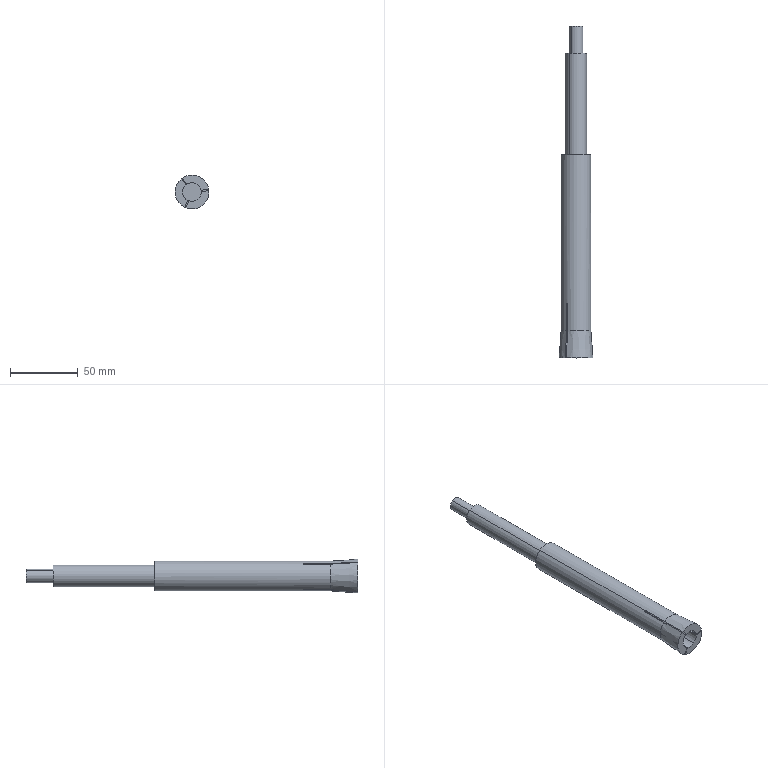Component | SolidWorks | HZ022-A001-D004-1 | 1 solid | 28 faces | box 25 x 245 x 25 mm | volume 51461 mm3 | plane 16 | cylinder 8 | cone 4 | commonest cylinder face diameters 10 x2 13.9 x2 22 x2 16 x2 | material S45C
STEP:
#1=COLOUR_RGB('',0.7922,0.8196,0.9333);
#2=FILL_AREA_STYLE_COLOUR('',#1);
#3=FILL_AREA_STYLE('',(#2));
#4=SURFACE_STYLE_FILL_AREA(#3);
#5=SURFACE_SIDE_STYLE('',(#4));
#6=SURFACE_STYLE_USAGE(.BOTH.,#5);
#7=PRESENTATION_STYLE_ASSIGNMENT((#6));
#8=CARTESIAN_POINT('',(-0.6243,0.2163,19.055));
#9=VERTEX_POINT('',#8);
#10=CARTESIAN_POINT('',(-0.3887,0.2163,18.74));
#11=VERTEX_POINT('',#10);
#12=CARTESIAN_POINT('',(-0.5065,0.2163,18.898));
#13=DIRECTION('',(0.,1.,0.));
#14=DIRECTION('',(-0.5984,0.,0.8012));
#15=AXIS2_PLACEMENT_3D('',#12,#13,#14);
#16=CIRCLE('',#15,0.1969);
#17=EDGE_CURVE('',#9,#11,#16,.T.);
#18=ORIENTED_EDGE('',*,*,#17,.T.);
#19=CARTESIAN_POINT('',(-0.3887,1.004,18.74));
#20=VERTEX_POINT('',#19);
#21=CARTESIAN_POINT('',(-0.3887,0.2163,18.74));
#22=DIRECTION('',(0.,1.,0.));
#23=VECTOR('',#22,39.37);
#24=LINE('',#21,#23);
#25=EDGE_CURVE('',#11,#20,#24,.T.);
#26=ORIENTED_EDGE('',*,*,#25,.T.);
#27=CARTESIAN_POINT('',(-0.6243,1.004,19.055));
#28=VERTEX_POINT('',#27);
#29=CARTESIAN_POINT('',(-0.5065,1.004,18.898));
#30=DIRECTION('',(0.,1.,0.));
#31=DIRECTION('',(-0.5984,0.,0.8012));
#32=AXIS2_PLACEMENT_3D('',#29,#30,#31);
#33=CIRCLE('',#32,0.1969);
#34=EDGE_CURVE('',#28,#20,#33,.T.);
#35=ORIENTED_EDGE('',*,*,#34,.F.);
#36=CARTESIAN_POINT('',(-0.6243,0.2163,19.055));
#37=DIRECTION('',(0.,1.,0.));
#38=VECTOR('',#37,39.37);
#39=LINE('',#36,#38);
#40=EDGE_CURVE('',#9,#28,#39,.T.);
#41=ORIENTED_EDGE('',*,*,#40,.F.);
#42=EDGE_LOOP('',(#18,#26,#35,#41));
#43=FACE_OUTER_BOUND('',#42,.T.);
#44=CARTESIAN_POINT('',(-0.5065,0.2163,18.898));
#45=DIRECTION('',(0.,1.,0.));
#46=DIRECTION('',(-0.5984,0.,0.8012));
#47=AXIS2_PLACEMENT_3D('',#44,#45,#46);
#48=CYLINDRICAL_SURFACE('',#47,0.1969);
#49=ADVANCED_FACE('',(#43),#48,.T.);
#50=CARTESIAN_POINT('',(-0.6702,-2.736,19.117));
#51=VERTEX_POINT('',#50);
#52=CARTESIAN_POINT('',(-0.3427,-2.736,18.678));
#53=VERTEX_POINT('',#52);
#54=CARTESIAN_POINT('',(-0.5065,-2.736,18.898));
#55=DIRECTION('',(0.,-1.,0.));
#56=DIRECTION('',(0.5984,0.,-0.8012));
#57=AXIS2_PLACEMENT_3D('',#54,#55,#56);
#58=CIRCLE('',#57,0.2736);
#59=EDGE_CURVE('',#51,#53,#58,.T.);
#60=ORIENTED_EDGE('',*,*,#59,.F.);
#61=CARTESIAN_POINT('',(-0.6702,-7.067,19.117));
#62=VERTEX_POINT('',#61);
#63=CARTESIAN_POINT('',(-0.6702,-2.736,19.117));
#64=DIRECTION('',(0.,-1.,0.));
#65=VECTOR('',#64,39.37);
#66=LINE('',#63,#65);
#67=EDGE_CURVE('',#51,#62,#66,.T.);
#68=ORIENTED_EDGE('',*,*,#67,.T.);
#69=CARTESIAN_POINT('',(-0.6856,-7.067,19.105));
#70=VERTEX_POINT('',#69);
#71=CARTESIAN_POINT('',(-0.5065,-7.067,18.898));
#72=DIRECTION('',(0.,1.,0.));
#73=DIRECTION('',(0.5984,0.,-0.8012));
#74=AXIS2_PLACEMENT_3D('',#71,#72,#73);
#75=CIRCLE('',#74,0.2736);
#76=EDGE_CURVE('',#70,#62,#75,.T.);
#77=ORIENTED_EDGE('',*,*,#76,.F.);
#78=CARTESIAN_POINT('',(-0.6856,-8.642,19.105));
#79=VERTEX_POINT('',#78);
#80=CARTESIAN_POINT('',(-0.6856,-2.736,19.105));
#81=DIRECTION('',(0.,-1.,0.));
#82=VECTOR('',#81,39.37);
#83=LINE('',#80,#82);
#84=EDGE_CURVE('',#70,#79,#83,.T.);
#85=ORIENTED_EDGE('',*,*,#84,.T.);
#86=CARTESIAN_POINT('',(-0.6323,-8.642,18.655));
#87=VERTEX_POINT('',#86);
#88=CARTESIAN_POINT('',(-0.5065,-8.642,18.898));
#89=DIRECTION('',(0.,-1.,0.));
#90=DIRECTION('',(0.5984,0.,-0.8012));
#91=AXIS2_PLACEMENT_3D('',#88,#89,#90);
#92=CIRCLE('',#91,0.2736);
#93=EDGE_CURVE('',#79,#87,#92,.T.);
#94=ORIENTED_EDGE('',*,*,#93,.T.);
#95=CARTESIAN_POINT('',(-0.6323,-7.067,18.655));
#96=VERTEX_POINT('',#95);
#97=CARTESIAN_POINT('',(-0.6323,-2.736,18.655));
#98=DIRECTION('',(0.,1.,0.));
#99=VECTOR('',#98,39.37);
#100=LINE('',#97,#99);
#101=EDGE_CURVE('',#87,#96,#100,.T.);
#102=ORIENTED_EDGE('',*,*,#101,.T.);
#103=CARTESIAN_POINT('',(-0.5961,-7.067,18.639));
#104=VERTEX_POINT('',#103);
#105=CARTESIAN_POINT('',(-0.5065,-7.067,18.898));
#106=DIRECTION('',(0.,1.,0.));
#107=DIRECTION('',(0.5984,0.,-0.8012));
#108=AXIS2_PLACEMENT_3D('',#105,#106,#107);
#109=CIRCLE('',#108,0.2736);
#110=EDGE_CURVE('',#104,#96,#109,.T.);
#111=ORIENTED_EDGE('',*,*,#110,.F.);
#112=CARTESIAN_POINT('',(-0.5961,-8.642,18.639));
#113=VERTEX_POINT('',#112);
#114=CARTESIAN_POINT('',(-0.5961,-2.736,18.639));
#115=DIRECTION('',(0.,-1.,0.));
#116=VECTOR('',#115,39.37);
#117=LINE('',#114,#116);
#118=EDGE_CURVE('',#104,#113,#117,.T.);
#119=ORIENTED_EDGE('',*,*,#118,.T.);
#120=CARTESIAN_POINT('',(-0.3427,-8.642,18.678));
#121=VERTEX_POINT('',#120);
#122=CARTESIAN_POINT('',(-0.5065,-8.642,18.898));
#123=DIRECTION('',(0.,-1.,0.));
#124=DIRECTION('',(0.5984,0.,-0.8012));
#125=AXIS2_PLACEMENT_3D('',#122,#123,#124);
#126=CIRCLE('',#125,0.2736);
#127=EDGE_CURVE('',#113,#121,#126,.T.);
#128=ORIENTED_EDGE('',*,*,#127,.T.);
#129=CARTESIAN_POINT('',(-0.3427,-2.736,18.678));
#130=DIRECTION('',(0.,-1.,0.));
#131=VECTOR('',#130,39.37);
#132=LINE('',#129,#131);
#133=EDGE_CURVE('',#53,#121,#132,.T.);
#134=ORIENTED_EDGE('',*,*,#133,.F.);
#135=EDGE_LOOP('',(#60,#68,#77,#85,#94,#102,#111,#119,#128,#134));
#136=FACE_OUTER_BOUND('',#135,.T.);
#137=CARTESIAN_POINT('',(-0.5065,-2.736,18.898));
#138=DIRECTION('',(0.,-1.,0.));
#139=DIRECTION('',(0.5984,0.,-0.8012));
#140=AXIS2_PLACEMENT_3D('',#137,#138,#139);
#141=CYLINDRICAL_SURFACE('',#140,0.2736);
#142=ADVANCED_FACE('',(#136),#141,.F.);
#143=CARTESIAN_POINT('',(-0.07456,-7.855,18.929));
#144=VERTEX_POINT('',#143);
#145=CARTESIAN_POINT('',(-0.2473,-7.855,18.551));
#146=VERTEX_POINT('',#145);
#147=CARTESIAN_POINT('',(-0.5065,-7.855,18.898));
#148=DIRECTION('',(0.,1.,0.));
#149=DIRECTION('',(-0.5984,0.,0.8012));
#150=AXIS2_PLACEMENT_3D('',#147,#148,#149);
#151=CIRCLE('',#150,0.4331);
#152=EDGE_CURVE('',#144,#146,#151,.T.);
#153=ORIENTED_EDGE('',*,*,#152,.T.);
#154=CARTESIAN_POINT('',(-0.2473,-2.736,18.551));
#155=VERTEX_POINT('',#154);
#156=CARTESIAN_POINT('',(-0.2473,-2.736,18.551));
#157=DIRECTION('',(0.,1.,0.));
#158=VECTOR('',#157,39.37);
#159=LINE('',#156,#158);
#160=EDGE_CURVE('',#146,#155,#159,.T.);
#161=ORIENTED_EDGE('',*,*,#160,.T.);
#162=CARTESIAN_POINT('',(-0.7657,-2.736,19.245));
#163=VERTEX_POINT('',#162);
#164=CARTESIAN_POINT('',(-0.5065,-2.736,18.898));
#165=DIRECTION('',(0.,1.,0.));
#166=DIRECTION('',(-0.5984,0.,0.8012));
#167=AXIS2_PLACEMENT_3D('',#164,#165,#166);
#168=CIRCLE('',#167,0.4331);
#169=EDGE_CURVE('',#163,#155,#168,.T.);
#170=ORIENTED_EDGE('',*,*,#169,.F.);
#171=CARTESIAN_POINT('',(-0.7657,-7.067,19.245));
#172=VERTEX_POINT('',#171);
#173=CARTESIAN_POINT('',(-0.7657,-2.736,19.245));
#174=DIRECTION('',(0.,1.,0.));
#175=VECTOR('',#174,39.37);
#176=LINE('',#173,#175);
#177=EDGE_CURVE('',#172,#163,#176,.T.);
#178=ORIENTED_EDGE('',*,*,#177,.F.);
#179=CARTESIAN_POINT('',(-0.7496,-7.067,19.256));
#180=VERTEX_POINT('',#179);
#181=CARTESIAN_POINT('',(-0.5065,-7.067,18.898));
#182=DIRECTION('',(0.,1.,0.));
#183=DIRECTION('',(0.5984,0.,-0.8012));
#184=AXIS2_PLACEMENT_3D('',#181,#182,#183);
#185=CIRCLE('',#184,0.4331);
#186=EDGE_CURVE('',#172,#180,#185,.T.);
#187=ORIENTED_EDGE('',*,*,#186,.T.);
#188=CARTESIAN_POINT('',(-0.7496,-7.855,19.256));
#189=VERTEX_POINT('',#188);
#190=CARTESIAN_POINT('',(-0.7496,-2.736,19.256));
#191=DIRECTION('',(0.,1.,0.));
#192=VECTOR('',#191,39.37);
#193=LINE('',#190,#192);
#194=EDGE_CURVE('',#189,#180,#193,.T.);
#195=ORIENTED_EDGE('',*,*,#194,.F.);
#196=CARTESIAN_POINT('',(-0.07919,-7.855,18.968));
#197=VERTEX_POINT('',#196);
#198=CARTESIAN_POINT('',(-0.5065,-7.855,18.898));
#199=DIRECTION('',(0.,1.,0.));
#200=DIRECTION('',(-0.5984,0.,0.8012));
#201=AXIS2_PLACEMENT_3D('',#198,#199,#200);
#202=CIRCLE('',#201,0.4331);
#203=EDGE_CURVE('',#189,#197,#202,.T.);
#204=ORIENTED_EDGE('',*,*,#203,.T.);
#205=CARTESIAN_POINT('',(-0.07919,-7.067,18.968));
#206=VERTEX_POINT('',#205);
#207=CARTESIAN_POINT('',(-0.07919,-2.736,18.968));
#208=DIRECTION('',(0.,-1.,0.));
#209=VECTOR('',#208,39.37);
#210=LINE('',#207,#209);
#211=EDGE_CURVE('',#206,#197,#210,.T.);
#212=ORIENTED_EDGE('',*,*,#211,.F.);
#213=CARTESIAN_POINT('',(-0.07456,-7.067,18.929));
#214=VERTEX_POINT('',#213);
#215=CARTESIAN_POINT('',(-0.5065,-7.067,18.898));
#216=DIRECTION('',(0.,1.,0.));
#217=DIRECTION('',(0.5984,0.,-0.8012));
#218=AXIS2_PLACEMENT_3D('',#215,#216,#217);
#219=CIRCLE('',#218,0.4331);
#220=EDGE_CURVE('',#206,#214,#219,.T.);
#221=ORIENTED_EDGE('',*,*,#220,.T.);
#222=CARTESIAN_POINT('',(-0.07456,-2.736,18.929));
#223=DIRECTION('',(0.,1.,0.));
#224=VECTOR('',#223,39.37);
#225=LINE('',#222,#224);
#226=EDGE_CURVE('',#144,#214,#225,.T.);
#227=ORIENTED_EDGE('',*,*,#226,.F.);
#228=EDGE_LOOP('',(#153,#161,#170,#178,#187,#195,#204,#212,#221,#227));
#229=FACE_OUTER_BOUND('',#228,.T.);
#230=CARTESIAN_POINT('',(-0.5065,-2.736,18.898));
#231=DIRECTION('',(0.,1.,0.));
#232=DIRECTION('',(-0.5984,0.,0.8012));
#233=AXIS2_PLACEMENT_3D('',#230,#231,#232);
#234=CYLINDRICAL_SURFACE('',#233,0.4331);
#235=ADVANCED_FACE('',(#229),#234,.T.);
#236=CARTESIAN_POINT('',(-0.6591,-7.855,18.492));
#237=VERTEX_POINT('',#236);
#238=CARTESIAN_POINT('',(-0.5065,-7.855,18.898));
#239=DIRECTION('',(0.,1.,0.));
#240=DIRECTION('',(-0.5984,0.,0.8012));
#241=AXIS2_PLACEMENT_3D('',#238,#239,#240);
#242=CIRCLE('',#241,0.4331);
#243=EDGE_CURVE('',#146,#237,#242,.T.);
#244=ORIENTED_EDGE('',*,*,#243,.F.);
#245=CARTESIAN_POINT('',(-0.212,-8.642,18.503));
#246=VERTEX_POINT('',#245);
#247=CARTESIAN_POINT('',(-0.2473,-7.855,18.551));
#248=DIRECTION('',(0.04476,-0.9972,-0.05992));
#249=VECTOR('',#248,39.37);
#250=LINE('',#247,#249);
#251=EDGE_CURVE('',#146,#246,#250,.T.);
#252=ORIENTED_EDGE('',*,*,#251,.T.);
#253=CARTESIAN_POINT('',(-0.6824,-8.642,18.438));
#254=VERTEX_POINT('',#253);
#255=CARTESIAN_POINT('',(-0.5065,-8.642,18.898));
#256=DIRECTION('',(0.,1.,0.));
#257=DIRECTION('',(-0.5984,0.,0.8012));
#258=AXIS2_PLACEMENT_3D('',#255,#256,#257);
#259=CIRCLE('',#258,0.4921);
#260=EDGE_CURVE('',#246,#254,#259,.T.);
#261=ORIENTED_EDGE('',*,*,#260,.T.);
#262=CARTESIAN_POINT('',(-0.6591,-7.855,18.492));
#263=CARTESIAN_POINT('',(-0.6669,-8.117,18.474));
#264=CARTESIAN_POINT('',(-0.6747,-8.379,18.456));
#265=CARTESIAN_POINT('',(-0.6824,-8.642,18.438));
#266=B_SPLINE_CURVE_WITH_KNOTS('',3,(#262,#263,#264,#265),.UNSPECIFIED.,.F.,.F.,(4,4),(0.0000002,0.02006),.UNSPECIFIED.);
#267=EDGE_CURVE('',#237,#254,#266,.T.);
#268=ORIENTED_EDGE('',*,*,#267,.F.);
#269=EDGE_LOOP('',(#244,#252,#261,#268));
#270=FACE_OUTER_BOUND('',#269,.T.);
#271=CARTESIAN_POINT('',(-0.5065,-7.855,18.898));
#272=DIRECTION('',(0.,-1.,0.));
#273=DIRECTION('',(0.5984,0.,-0.8012));
#274=AXIS2_PLACEMENT_3D('',#271,#272,#273);
#275=CONICAL_SURFACE('',#274,0.4331,0.07486);
#276=ADVANCED_FACE('',(#270),#275,.T.);
#277=CARTESIAN_POINT('',(-0.695,0.2163,19.15));
#278=VERTEX_POINT('',#277);
#279=CARTESIAN_POINT('',(-0.318,0.2163,18.645));
#280=VERTEX_POINT('',#279);
#281=CARTESIAN_POINT('',(-0.5065,0.2163,18.898));
#282=DIRECTION('',(0.,1.,0.));
#283=DIRECTION('',(-0.5984,0.,0.8012));
#284=AXIS2_PLACEMENT_3D('',#281,#282,#283);
#285=CIRCLE('',#284,0.315);
#286=EDGE_CURVE('',#278,#280,#285,.T.);
#287=ORIENTED_EDGE('',*,*,#286,.F.);
#288=CARTESIAN_POINT('',(-0.695,-2.736,19.15));
#289=VERTEX_POINT('',#288);
#290=CARTESIAN_POINT('',(-0.695,1.004,19.15));
#291=DIRECTION('',(0.,-1.,0.));
#292=VECTOR('',#291,39.37);
#293=LINE('',#290,#292);
#294=EDGE_CURVE('',#278,#289,#293,.T.);
#295=ORIENTED_EDGE('',*,*,#294,.T.);
#296=CARTESIAN_POINT('',(-0.318,-2.736,18.645));
#297=VERTEX_POINT('',#296);
#298=CARTESIAN_POINT('',(-0.5065,-2.736,18.898));
#299=DIRECTION('',(0.,1.,0.));
#300=DIRECTION('',(-0.5984,0.,0.8012));
#301=AXIS2_PLACEMENT_3D('',#298,#299,#300);
#302=CIRCLE('',#301,0.315);
#303=EDGE_CURVE('',#289,#297,#302,.T.);
#304=ORIENTED_EDGE('',*,*,#303,.T.);
#305=CARTESIAN_POINT('',(-0.318,1.004,18.645));
#306=DIRECTION('',(0.,-1.,0.));
#307=VECTOR('',#306,39.37);
#308=LINE('',#305,#307);
#309=EDGE_CURVE('',#280,#297,#308,.T.);
#310=ORIENTED_EDGE('',*,*,#309,.F.);
#311=EDGE_LOOP('',(#287,#295,#304,#310));
#312=FACE_OUTER_BOUND('',#311,.T.);
#313=CARTESIAN_POINT('',(-0.5065,1.004,18.898));
#314=DIRECTION('',(0.,-1.,0.));
#315=DIRECTION('',(0.5984,0.,-0.8012));
#316=AXIS2_PLACEMENT_3D('',#313,#314,#315);
#317=CYLINDRICAL_SURFACE('',#316,0.315);
#318=ADVANCED_FACE('',(#312),#317,.T.);
#319=ORIENTED_EDGE('',*,*,#294,.F.);
#320=CARTESIAN_POINT('',(-0.5065,0.2163,18.898));
#321=DIRECTION('',(0.,1.,0.));
#322=DIRECTION('',(-0.5984,0.,0.8012));
#323=AXIS2_PLACEMENT_3D('',#320,#321,#322);
#324=CIRCLE('',#323,0.315);
#325=EDGE_CURVE('',#280,#278,#324,.T.);
#326=ORIENTED_EDGE('',*,*,#325,.F.);
#327=ORIENTED_EDGE('',*,*,#309,.T.);
#328=CARTESIAN_POINT('',(-0.5065,-2.736,18.898));
#329=DIRECTION('',(0.,1.,0.));
#330=DIRECTION('',(-0.5984,0.,0.8012));
#331=AXIS2_PLACEMENT_3D('',#328,#329,#330);
#332=CIRCLE('',#331,0.315);
#333=EDGE_CURVE('',#297,#289,#332,.T.);
#334=ORIENTED_EDGE('',*,*,#333,.T.);
#335=EDGE_LOOP('',(#319,#326,#327,#334));
#336=FACE_OUTER_BOUND('',#335,.T.);
#337=CARTESIAN_POINT('',(-0.5065,1.004,18.898));
#338=DIRECTION('',(0.,-1.,0.));
#339=DIRECTION('',(0.5984,0.,-0.8012));
#340=AXIS2_PLACEMENT_3D('',#337,#338,#339);
#341=CYLINDRICAL_SURFACE('',#340,0.315);
#342=ADVANCED_FACE('',(#336),#341,.T.);
#343=CARTESIAN_POINT('',(-0.7186,-8.642,18.454));
#344=VERTEX_POINT('',#343);
#345=CARTESIAN_POINT('',(-0.9263,-8.642,17.97));
#346=DIRECTION('',(-0.3946,0.,-0.9188));
#347=VECTOR('',#346,39.37);
#348=LINE('',#345,#347);
#349=EDGE_CURVE('',#87,#344,#348,.T.);
#350=ORIENTED_EDGE('',*,*,#349,.F.);
#351=ORIENTED_EDGE('',*,*,#93,.F.);
#352=CARTESIAN_POINT('',(-0.8165,-8.642,19.28));
#353=VERTEX_POINT('',#352);
#354=CARTESIAN_POINT('',(-1.131,-8.642,19.701));
#355=DIRECTION('',(0.5984,0.,-0.8012));
#356=VECTOR('',#355,39.37);
#357=LINE('',#354,#356);
#358=EDGE_CURVE('',#353,#79,#357,.T.);
#359=ORIENTED_EDGE('',*,*,#358,.F.);
#360=CARTESIAN_POINT('',(-0.5065,-8.642,18.898));
#361=DIRECTION('',(0.,1.,0.));
#362=DIRECTION('',(-0.5984,0.,0.8012));
#363=AXIS2_PLACEMENT_3D('',#360,#361,#362);
#364=CIRCLE('',#363,0.4921);
#365=EDGE_CURVE('',#344,#353,#364,.T.);
#366=ORIENTED_EDGE('',*,*,#365,.F.);
#367=EDGE_LOOP('',(#350,#351,#359,#366));
#368=FACE_OUTER_BOUND('',#367,.T.);
#369=CARTESIAN_POINT('',(-0.5065,-8.642,18.898));
#370=DIRECTION('',(0.,-1.,0.));
#371=DIRECTION('',(0.5984,0.,-0.8012));
#372=AXIS2_PLACEMENT_3D('',#369,#370,#371);
#373=PLANE('',#372);
#374=ADVANCED_FACE('',(#368),#373,.T.);
#375=CARTESIAN_POINT('',(-0.0205,-8.642,18.975));
#376=VERTEX_POINT('',#375);
#377=CARTESIAN_POINT('',(-0.2378,-8.642,18.949));
#378=VERTEX_POINT('',#377);
#379=CARTESIAN_POINT('',(0.5021,-8.642,19.037));
#380=DIRECTION('',(-0.9931,0.,-0.1177));
#381=VECTOR('',#380,39.37);
#382=LINE('',#379,#381);
#383=EDGE_CURVE('',#376,#378,#382,.T.);
#384=ORIENTED_EDGE('',*,*,#383,.F.);
#385=CARTESIAN_POINT('',(-0.785,-8.642,19.303));
#386=VERTEX_POINT('',#385);
#387=CARTESIAN_POINT('',(-0.5065,-8.642,18.898));
#388=DIRECTION('',(0.,1.,0.));
#389=DIRECTION('',(-0.5984,0.,0.8012));
#390=AXIS2_PLACEMENT_3D('',#387,#388,#389);
#391=CIRCLE('',#390,0.4921);
#392=EDGE_CURVE('',#386,#376,#391,.T.);
#393=ORIENTED_EDGE('',*,*,#392,.F.);
#394=CARTESIAN_POINT('',(-0.654,-8.642,19.128));
#395=VERTEX_POINT('',#394);
#396=CARTESIAN_POINT('',(-1.1,-8.642,19.725));
#397=DIRECTION('',(-0.5984,0.,0.8012));
#398=VECTOR('',#397,39.37);
#399=LINE('',#396,#398);
#400=EDGE_CURVE('',#395,#386,#399,.T.);
#401=ORIENTED_EDGE('',*,*,#400,.F.);
#402=CARTESIAN_POINT('',(-0.5065,-8.642,18.898));
#403=DIRECTION('',(0.,-1.,0.));
#404=DIRECTION('',(0.5984,0.,-0.8012));
#405=AXIS2_PLACEMENT_3D('',#402,#403,#404);
#406=CIRCLE('',#405,0.2736);
#407=EDGE_CURVE('',#378,#395,#406,.T.);
#408=ORIENTED_EDGE('',*,*,#407,.F.);
#409=EDGE_LOOP('',(#384,#393,#401,#408));
#410=FACE_OUTER_BOUND('',#409,.T.);
#411=CARTESIAN_POINT('',(-0.5065,-8.642,18.898));
#412=DIRECTION('',(0.,-1.,0.));
#413=DIRECTION('',(0.5984,0.,-0.8012));
#414=AXIS2_PLACEMENT_3D('',#411,#412,#413);
#415=PLANE('',#414);
#416=ADVANCED_FACE('',(#410),#415,.T.);
#417=CARTESIAN_POINT('',(-0.6953,-7.855,18.508));
#418=VERTEX_POINT('',#417);
#419=CARTESIAN_POINT('',(-0.7186,-8.642,18.454));
#420=CARTESIAN_POINT('',(-0.7108,-8.379,18.472));
#421=CARTESIAN_POINT('',(-0.7031,-8.117,18.49));
#422=CARTESIAN_POINT('',(-0.6953,-7.855,18.508));
#423=B_SPLINE_CURVE_WITH_KNOTS('',3,(#419,#420,#421,#422),.UNSPECIFIED.,.F.,.F.,(4,4),(0.0000002,0.02006),.UNSPECIFIED.);
#424=EDGE_CURVE('',#344,#418,#423,.T.);
#425=ORIENTED_EDGE('',*,*,#424,.F.);
#426=ORIENTED_EDGE('',*,*,#365,.T.);
#427=CARTESIAN_POINT('',(-0.7812,-7.855,19.232));
#428=VERTEX_POINT('',#427);
#429=CARTESIAN_POINT('',(-0.7812,-7.855,19.232));
#430=CARTESIAN_POINT('',(-0.7826,-7.885,19.234));
#431=CARTESIAN_POINT('',(-0.7839,-7.916,19.236));
#432=CARTESIAN_POINT('',(-0.7853,-7.947,19.238));
#433=CARTESIAN_POINT('',(-0.7957,-8.179,19.252));
#434=CARTESIAN_POINT('',(-0.8061,-8.41,19.266));
#435=CARTESIAN_POINT('',(-0.8165,-8.642,19.28));
#436=B_SPLINE_CURVE_WITH_KNOTS('',3,(#429,#430,#431,#432,#433,#434,#435),.UNSPECIFIED.,.F.,.F.,(4,3,4),(0.01844,0.0208,0.0385),.UNSPECIFIED.);
#437=EDGE_CURVE('',#428,#353,#436,.T.);
#438=ORIENTED_EDGE('',*,*,#437,.F.);
#439=CARTESIAN_POINT('',(-0.5065,-7.855,18.898));
#440=DIRECTION('',(0.,1.,0.));
#441=DIRECTION('',(-0.5984,0.,0.8012));
#442=AXIS2_PLACEMENT_3D('',#439,#440,#441);
#443=CIRCLE('',#442,0.4331);
#444=EDGE_CURVE('',#418,#428,#443,.T.);
#445=ORIENTED_EDGE('',*,*,#444,.F.);
#446=EDGE_LOOP('',(#425,#426,#438,#445));
#447=FACE_OUTER_BOUND('',#446,.T.);
#448=CARTESIAN_POINT('',(-0.5065,-7.855,18.898));
#449=DIRECTION('',(0.,-1.,0.));
#450=DIRECTION('',(0.5984,0.,-0.8012));
#451=AXIS2_PLACEMENT_3D('',#448,#449,#450);
#452=CONICAL_SURFACE('',#451,0.4331,0.07486);
#453=ADVANCED_FACE('',(#447),#452,.T.);
#454=CARTESIAN_POINT('',(-0.07919,-7.855,18.968));
#455=CARTESIAN_POINT('',(-0.05963,-8.117,18.97));
#456=CARTESIAN_POINT('',(-0.04006,-8.379,18.973));
#457=CARTESIAN_POINT('',(-0.0205,-8.642,18.975));
#458=B_SPLINE_CURVE_WITH_KNOTS('',3,(#454,#455,#456,#457),.UNSPECIFIED.,.F.,.F.,(4,4),(0.0000002,0.02006),.UNSPECIFIED.);
#459=EDGE_CURVE('',#197,#376,#458,.T.);
#460=ORIENTED_EDGE('',*,*,#459,.F.);
#461=ORIENTED_EDGE('',*,*,#203,.F.);
#462=CARTESIAN_POINT('',(-0.785,-8.642,19.303));
#463=CARTESIAN_POINT('',(-0.7746,-8.41,19.289));
#464=CARTESIAN_POINT('',(-0.7642,-8.179,19.276));
#465=CARTESIAN_POINT('',(-0.7538,-7.947,19.262));
#466=CARTESIAN_POINT('',(-0.7524,-7.916,19.26));
#467=CARTESIAN_POINT('',(-0.751,-7.885,19.258));
#468=CARTESIAN_POINT('',(-0.7496,-7.855,19.256));
#469=B_SPLINE_CURVE_WITH_KNOTS('',3,(#462,#463,#464,#465,#466,#467,#468),.UNSPECIFIED.,.F.,.F.,(4,3,4),(0.04955,0.06725,0.0696),.UNSPECIFIED.);
#470=EDGE_CURVE('',#386,#189,#469,.T.);
#471=ORIENTED_EDGE('',*,*,#470,.F.);
#472=ORIENTED_EDGE('',*,*,#392,.T.);
#473=EDGE_LOOP('',(#460,#461,#471,#472));
#474=FACE_OUTER_BOUND('',#473,.T.);
#475=CARTESIAN_POINT('',(-0.5065,-7.855,18.898));
#476=DIRECTION('',(0.,-1.,0.));
#477=DIRECTION('',(0.5984,0.,-0.8012));
#478=AXIS2_PLACEMENT_3D('',#475,#476,#477);
#479=CONICAL_SURFACE('',#478,0.4331,0.07486);
#480=ADVANCED_FACE('',(#474),#479,.T.);
#481=ORIENTED_EDGE('',*,*,#333,.F.);
#482=ORIENTED_EDGE('',*,*,#303,.F.);
#483=EDGE_LOOP('',(#481,#482));
#484=FACE_BOUND('',#483,.T.);
#485=ORIENTED_EDGE('',*,*,#169,.T.);
#486=CARTESIAN_POINT('',(-0.5065,-2.736,18.898));
#487=DIRECTION('',(0.,1.,0.));
#488=DIRECTION('',(-0.5984,0.,0.8012));
#489=AXIS2_PLACEMENT_3D('',#486,#487,#488);
#490=CIRCLE('',#489,0.4331);
#491=EDGE_CURVE('',#155,#163,#490,.T.);
#492=ORIENTED_EDGE('',*,*,#491,.T.);
#493=EDGE_LOOP('',(#485,#492));
#494=FACE_OUTER_BOUND('',#493,.T.);
#495=CARTESIAN_POINT('',(-0.7657,-2.736,19.245));
#496=DIRECTION('',(0.,1.,0.));
#497=DIRECTION('',(-0.5984,0.,0.8012));
#498=AXIS2_PLACEMENT_3D('',#495,#496,#497);
#499=PLANE('',#498);
#500=ADVANCED_FACE('',(#484,#494),#499,.T.);
#501=CARTESIAN_POINT('',(-0.8901,-8.642,17.955));
#502=DIRECTION('',(0.3946,0.,0.9188));
#503=VECTOR('',#502,39.37);
#504=LINE('',#501,#503);
#505=EDGE_CURVE('',#254,#113,#504,.T.);
#506=ORIENTED_EDGE('',*,*,#505,.F.);
#507=ORIENTED_EDGE('',*,*,#260,.F.);
#508=CARTESIAN_POINT('',(-0.01586,-8.642,18.936));
#509=VERTEX_POINT('',#508);
#510=CARTESIAN_POINT('',(-0.5065,-8.642,18.898));
#511=DIRECTION('',(0.,1.,0.));
#512=DIRECTION('',(-0.5984,0.,0.8012));
#513=AXIS2_PLACEMENT_3D('',#510,#511,#512);
#514=CIRCLE('',#513,0.4921);
#515=EDGE_CURVE('',#509,#246,#514,.T.);
#516=ORIENTED_EDGE('',*,*,#515,.F.);
#517=CARTESIAN_POINT('',(-0.2332,-8.642,18.91));
#518=VERTEX_POINT('',#517);
#519=CARTESIAN_POINT('',(0.5067,-8.642,18.998));
#520=DIRECTION('',(0.9931,0.,0.1177));
#521=VECTOR('',#520,39.37);
#522=LINE('',#519,#521);
#523=EDGE_CURVE('',#518,#509,#522,.T.);
#524=ORIENTED_EDGE('',*,*,#523,.F.);
#525=CARTESIAN_POINT('',(-0.5065,-8.642,18.898));
#526=DIRECTION('',(0.,-1.,0.));
#527=DIRECTION('',(0.5984,0.,-0.8012));
#528=AXIS2_PLACEMENT_3D('',#525,#526,#527);
#529=CIRCLE('',#528,0.2736);
#530=EDGE_CURVE('',#121,#518,#529,.T.);
#531=ORIENTED_EDGE('',*,*,#530,.F.);
#532=ORIENTED_EDGE('',*,*,#127,.F.);
#533=EDGE_LOOP('',(#506,#507,#516,#524,#531,#532));
#534=FACE_OUTER_BOUND('',#533,.T.);
#535=CARTESIAN_POINT('',(-0.5065,-8.642,18.898));
#536=DIRECTION('',(0.,-1.,0.));
#537=DIRECTION('',(0.5984,0.,-0.8012));
#538=AXIS2_PLACEMENT_3D('',#535,#536,#537);
#539=PLANE('',#538);
#540=ADVANCED_FACE('',(#534),#539,.T.);
#541=ORIENTED_EDGE('',*,*,#251,.F.);
#542=ORIENTED_EDGE('',*,*,#152,.F.);
#543=CARTESIAN_POINT('',(-0.01586,-8.642,18.936));
#544=CARTESIAN_POINT('',(-0.03543,-8.379,18.934));
#545=CARTESIAN_POINT('',(-0.05499,-8.117,18.931));
#546=CARTESIAN_POINT('',(-0.07456,-7.855,18.929));
#547=B_SPLINE_CURVE_WITH_KNOTS('',3,(#543,#544,#545,#546),.UNSPECIFIED.,.F.,.F.,(4,4),(0.0000002,0.02006),.UNSPECIFIED.);
#548=EDGE_CURVE('',#509,#144,#547,.T.);
#549=ORIENTED_EDGE('',*,*,#548,.F.);
#550=ORIENTED_EDGE('',*,*,#515,.T.);
#551=EDGE_LOOP('',(#541,#542,#549,#550));
#552=FACE_OUTER_BOUND('',#551,.T.);
#553=CARTESIAN_POINT('',(-0.5065,-7.855,18.898));
#554=DIRECTION('',(0.,-1.,0.));
#555=DIRECTION('',(0.5984,0.,-0.8012));
#556=AXIS2_PLACEMENT_3D('',#553,#554,#555);
#557=CONICAL_SURFACE('',#556,0.4331,0.07486);
#558=ADVANCED_FACE('',(#552),#557,.T.);
#559=ORIENTED_EDGE('',*,*,#160,.F.);
#560=ORIENTED_EDGE('',*,*,#243,.T.);
#561=CARTESIAN_POINT('',(-0.6591,-7.067,18.492));
#562=VERTEX_POINT('',#561);
#563=CARTESIAN_POINT('',(-0.6591,-2.736,18.492));
#564=DIRECTION('',(0.,-1.,0.));
#565=VECTOR('',#564,39.37);
#566=LINE('',#563,#565);
#567=EDGE_CURVE('',#562,#237,#566,.T.);
#568=ORIENTED_EDGE('',*,*,#567,.F.);
#569=CARTESIAN_POINT('',(-0.6953,-7.067,18.508));
#570=VERTEX_POINT('',#569);
#571=CARTESIAN_POINT('',(-0.5065,-7.067,18.898));
#572=DIRECTION('',(0.,1.,0.));
#573=DIRECTION('',(0.5984,0.,-0.8012));
#574=AXIS2_PLACEMENT_3D('',#571,#572,#573);
#575=CIRCLE('',#574,0.4331);
#576=EDGE_CURVE('',#562,#570,#575,.T.);
#577=ORIENTED_EDGE('',*,*,#576,.T.);
#578=CARTESIAN_POINT('',(-0.6953,-2.736,18.508));
#579=DIRECTION('',(0.,1.,0.));
#580=VECTOR('',#579,39.37);
#581=LINE('',#578,#580);
#582=EDGE_CURVE('',#418,#570,#581,.T.);
#583=ORIENTED_EDGE('',*,*,#582,.F.);
#584=ORIENTED_EDGE('',*,*,#444,.T.);
#585=CARTESIAN_POINT('',(-0.7812,-7.067,19.232));
#586=VERTEX_POINT('',#585);
#587=CARTESIAN_POINT('',(-0.7812,-2.736,19.232));
#588=DIRECTION('',(0.,-1.,0.));
#589=VECTOR('',#588,39.37);
#590=LINE('',#587,#589);
#591=EDGE_CURVE('',#586,#428,#590,.T.);
#592=ORIENTED_EDGE('',*,*,#591,.F.);
#593=CARTESIAN_POINT('',(-0.5065,-7.067,18.898));
#594=DIRECTION('',(0.,1.,0.));
#595=DIRECTION('',(0.5984,0.,-0.8012));
#596=AXIS2_PLACEMENT_3D('',#593,#594,#595);
#597=CIRCLE('',#596,0.4331);
#598=EDGE_CURVE('',#586,#172,#597,.T.);
#599=ORIENTED_EDGE('',*,*,#598,.T.);
#600=ORIENTED_EDGE('',*,*,#177,.T.);
#601=ORIENTED_EDGE('',*,*,#491,.F.);
#602=EDGE_LOOP('',(#559,#560,#568,#577,#583,#584,#592,#599,#600,#601));
#603=FACE_OUTER_BOUND('',#602,.T.);
#604=CARTESIAN_POINT('',(-0.5065,-2.736,18.898));
#605=DIRECTION('',(0.,1.,0.));
#606=DIRECTION('',(-0.5984,0.,0.8012));
#607=AXIS2_PLACEMENT_3D('',#604,#605,#606);
#608=CYLINDRICAL_SURFACE('',#607,0.4331);
#609=ADVANCED_FACE('',(#603),#608,.T.);
#610=ORIENTED_EDGE('',*,*,#67,.F.);
#611=CARTESIAN_POINT('',(-0.5065,-2.736,18.898));
#612=DIRECTION('',(0.,-1.,0.));
#613=DIRECTION('',(0.5984,0.,-0.8012));
#614=AXIS2_PLACEMENT_3D('',#611,#612,#613);
#615=CIRCLE('',#614,0.2736);
#616=EDGE_CURVE('',#53,#51,#615,.T.);
#617=ORIENTED_EDGE('',*,*,#616,.F.);
#618=ORIENTED_EDGE('',*,*,#133,.T.);
#619=ORIENTED_EDGE('',*,*,#530,.T.);
#620=CARTESIAN_POINT('',(-0.2332,-7.067,18.91));
#621=VERTEX_POINT('',#620);
#622=CARTESIAN_POINT('',(-0.2332,-2.736,18.91));
#623=DIRECTION('',(0.,1.,0.));
#624=VECTOR('',#623,39.37);
#625=LINE('',#622,#624);
#626=EDGE_CURVE('',#518,#621,#625,.T.);
#627=ORIENTED_EDGE('',*,*,#626,.T.);
#628=CARTESIAN_POINT('',(-0.2378,-7.067,18.949));
#629=VERTEX_POINT('',#628);
#630=CARTESIAN_POINT('',(-0.5065,-7.067,18.898));
#631=DIRECTION('',(0.,1.,0.));
#632=DIRECTION('',(0.5984,0.,-0.8012));
#633=AXIS2_PLACEMENT_3D('',#630,#631,#632);
#634=CIRCLE('',#633,0.2736);
#635=EDGE_CURVE('',#629,#621,#634,.T.);
#636=ORIENTED_EDGE('',*,*,#635,.F.);
#637=CARTESIAN_POINT('',(-0.2378,-2.736,18.949));
#638=DIRECTION('',(0.,-1.,0.));
#639=VECTOR('',#638,39.37);
#640=LINE('',#637,#639);
#641=EDGE_CURVE('',#629,#378,#640,.T.);
#642=ORIENTED_EDGE('',*,*,#641,.T.);
#643=ORIENTED_EDGE('',*,*,#407,.T.);
#644=CARTESIAN_POINT('',(-0.654,-7.067,19.128));
#645=VERTEX_POINT('',#644);
#646=CARTESIAN_POINT('',(-0.654,-2.736,19.128));
#647=DIRECTION('',(0.,1.,0.));
#648=VECTOR('',#647,39.37);
#649=LINE('',#646,#648);
#650=EDGE_CURVE('',#395,#645,#649,.T.);
#651=ORIENTED_EDGE('',*,*,#650,.T.);
#652=CARTESIAN_POINT('',(-0.5065,-7.067,18.898));
#653=DIRECTION('',(0.,1.,0.));
#654=DIRECTION('',(0.5984,0.,-0.8012));
#655=AXIS2_PLACEMENT_3D('',#652,#653,#654);
#656=CIRCLE('',#655,0.2736);
#657=EDGE_CURVE('',#62,#645,#656,.T.);
#658=ORIENTED_EDGE('',*,*,#657,.F.);
#659=EDGE_LOOP('',(#610,#617,#618,#619,#627,#636,#642,#643,#651,#658));
#660=FACE_OUTER_BOUND('',#659,.T.);
#661=CARTESIAN_POINT('',(-0.5065,-2.736,18.898));
#662=DIRECTION('',(0.,-1.,0.));
#663=DIRECTION('',(0.5984,0.,-0.8012));
#664=AXIS2_PLACEMENT_3D('',#661,#662,#663);
#665=CYLINDRICAL_SURFACE('',#664,0.2736);
#666=ADVANCED_FACE('',(#660),#665,.F.);
#667=ORIENTED_EDGE('',*,*,#470,.T.);
#668=ORIENTED_EDGE('',*,*,#194,.T.);
#669=CARTESIAN_POINT('',(-1.1,-7.067,19.725));
#670=DIRECTION('',(-0.5984,0.,0.8012));
#671=VECTOR('',#670,39.37);
#672=LINE('',#669,#671);
#673=EDGE_CURVE('',#645,#180,#672,.T.);
#674=ORIENTED_EDGE('',*,*,#673,.F.);
#675=ORIENTED_EDGE('',*,*,#650,.F.);
#676=ORIENTED_EDGE('',*,*,#400,.T.);
#677=EDGE_LOOP('',(#667,#668,#674,#675,#676));
#678=FACE_OUTER_BOUND('',#677,.T.);
#679=CARTESIAN_POINT('',(-1.1,-7.067,19.725));
#680=DIRECTION('',(0.8012,0.,0.5984));
#681=DIRECTION('',(-0.5984,0.,0.8012));
#682=AXIS2_PLACEMENT_3D('',#679,#680,#681);
#683=PLANE('',#682);
#684=ADVANCED_FACE('',(#678),#683,.F.);
#685=ORIENTED_EDGE('',*,*,#437,.T.);
#686=ORIENTED_EDGE('',*,*,#358,.T.);
#687=ORIENTED_EDGE('',*,*,#84,.F.);
#688=CARTESIAN_POINT('',(-1.131,-7.067,19.701));
#689=DIRECTION('',(0.5984,0.,-0.8012));
#690=VECTOR('',#689,39.37);
#691=LINE('',#688,#690);
#692=EDGE_CURVE('',#586,#70,#691,.T.);
#693=ORIENTED_EDGE('',*,*,#692,.F.);
#694=ORIENTED_EDGE('',*,*,#591,.T.);
#695=EDGE_LOOP('',(#685,#686,#687,#693,#694));
#696=FACE_OUTER_BOUND('',#695,.T.);
#697=CARTESIAN_POINT('',(-1.131,-7.067,19.701));
#698=DIRECTION('',(-0.8012,0.,-0.5984));
#699=DIRECTION('',(0.5984,0.,-0.8012));
#700=AXIS2_PLACEMENT_3D('',#697,#698,#699);
#701=PLANE('',#700);
#702=ADVANCED_FACE('',(#696),#701,.F.);
#703=ORIENTED_EDGE('',*,*,#692,.T.);
#704=ORIENTED_EDGE('',*,*,#76,.T.);
#705=ORIENTED_EDGE('',*,*,#657,.T.);
#706=ORIENTED_EDGE('',*,*,#673,.T.);
#707=ORIENTED_EDGE('',*,*,#186,.F.);
#708=ORIENTED_EDGE('',*,*,#598,.F.);
#709=EDGE_LOOP('',(#703,#704,#705,#706,#707,#708));
#710=FACE_OUTER_BOUND('',#709,.T.);
#711=CARTESIAN_POINT('',(-0.5065,-7.067,18.898));
#712=DIRECTION('',(0.,-1.,0.));
#713=DIRECTION('',(0.5984,0.,-0.8012));
#714=AXIS2_PLACEMENT_3D('',#711,#712,#713);
#715=PLANE('',#714);
#716=ADVANCED_FACE('',(#710),#715,.T.);
#717=ORIENTED_EDGE('',*,*,#548,.T.);
#718=ORIENTED_EDGE('',*,*,#226,.T.);
#719=CARTESIAN_POINT('',(0.5067,-7.067,18.998));
#720=DIRECTION('',(0.9931,0.,0.1177));
#721=VECTOR('',#720,39.37);
#722=LINE('',#719,#721);
#723=EDGE_CURVE('',#621,#214,#722,.T.);
#724=ORIENTED_EDGE('',*,*,#723,.F.);
#725=ORIENTED_EDGE('',*,*,#626,.F.);
#726=ORIENTED_EDGE('',*,*,#523,.T.);
#727=EDGE_LOOP('',(#717,#718,#724,#725,#726));
#728=FACE_OUTER_BOUND('',#727,.T.);
#729=CARTESIAN_POINT('',(0.5067,-7.067,18.998));
#730=DIRECTION('',(0.1177,0.,-0.9931));
#731=DIRECTION('',(0.9931,0.,0.1177));
#732=AXIS2_PLACEMENT_3D('',#729,#730,#731);
#733=PLANE('',#732);
#734=ADVANCED_FACE('',(#728),#733,.F.);
#735=ORIENTED_EDGE('',*,*,#459,.T.);
#736=ORIENTED_EDGE('',*,*,#383,.T.);
#737=ORIENTED_EDGE('',*,*,#641,.F.);
#738=CARTESIAN_POINT('',(0.5021,-7.067,19.037));
#739=DIRECTION('',(-0.9931,0.,-0.1177));
#740=VECTOR('',#739,39.37);
#741=LINE('',#738,#740);
#742=EDGE_CURVE('',#206,#629,#741,.T.);
#743=ORIENTED_EDGE('',*,*,#742,.F.);
#744=ORIENTED_EDGE('',*,*,#211,.T.);
#745=EDGE_LOOP('',(#735,#736,#737,#743,#744));
#746=FACE_OUTER_BOUND('',#745,.T.);
#747=CARTESIAN_POINT('',(0.5021,-7.067,19.037));
#748=DIRECTION('',(-0.1177,0.,0.9931));
#749=DIRECTION('',(-0.9931,0.,-0.1177));
#750=AXIS2_PLACEMENT_3D('',#747,#748,#749);
#751=PLANE('',#750);
#752=ADVANCED_FACE('',(#746),#751,.F.);
#753=ORIENTED_EDGE('',*,*,#742,.T.);
#754=ORIENTED_EDGE('',*,*,#635,.T.);
#755=ORIENTED_EDGE('',*,*,#723,.T.);
#756=ORIENTED_EDGE('',*,*,#220,.F.);
#757=EDGE_LOOP('',(#753,#754,#755,#756));
#758=FACE_OUTER_BOUND('',#757,.T.);
#759=CARTESIAN_POINT('',(-0.5065,-7.067,18.898));
#760=DIRECTION('',(0.,-1.,0.));
#761=DIRECTION('',(0.3946,0.,0.9188));
#762=AXIS2_PLACEMENT_3D('',#759,#760,#761);
#763=PLANE('',#762);
#764=ADVANCED_FACE('',(#758),#763,.T.);
#765=ORIENTED_EDGE('',*,*,#424,.T.);
#766=ORIENTED_EDGE('',*,*,#582,.T.);
#767=CARTESIAN_POINT('',(-0.9263,-7.067,17.97));
#768=DIRECTION('',(-0.3946,0.,-0.9188));
#769=VECTOR('',#768,39.37);
#770=LINE('',#767,#769);
#771=EDGE_CURVE('',#96,#570,#770,.T.);
#772=ORIENTED_EDGE('',*,*,#771,.F.);
#773=ORIENTED_EDGE('',*,*,#101,.F.);
#774=ORIENTED_EDGE('',*,*,#349,.T.);
#775=EDGE_LOOP('',(#765,#766,#772,#773,#774));
#776=FACE_OUTER_BOUND('',#775,.T.);
#777=CARTESIAN_POINT('',(-0.9263,-7.067,17.97));
#778=DIRECTION('',(-0.9188,0.,0.3946));
#779=DIRECTION('',(-0.3946,0.,-0.9188));
#780=AXIS2_PLACEMENT_3D('',#777,#778,#779);
#781=PLANE('',#780);
#782=ADVANCED_FACE('',(#776),#781,.F.);
#783=ORIENTED_EDGE('',*,*,#267,.T.);
#784=ORIENTED_EDGE('',*,*,#505,.T.);
#785=ORIENTED_EDGE('',*,*,#118,.F.);
#786=CARTESIAN_POINT('',(-0.8901,-7.067,17.955));
#787=DIRECTION('',(0.3946,0.,0.9188));
#788=VECTOR('',#787,39.37);
#789=LINE('',#786,#788);
#790=EDGE_CURVE('',#562,#104,#789,.T.);
#791=ORIENTED_EDGE('',*,*,#790,.F.);
#792=ORIENTED_EDGE('',*,*,#567,.T.);
#793=EDGE_LOOP('',(#783,#784,#785,#791,#792));
#794=FACE_OUTER_BOUND('',#793,.T.);
#795=CARTESIAN_POINT('',(-0.8901,-7.067,17.955));
#796=DIRECTION('',(0.9188,0.,-0.3946));
#797=DIRECTION('',(0.3946,0.,0.9188));
#798=AXIS2_PLACEMENT_3D('',#795,#796,#797);
#799=PLANE('',#798);
#800=ADVANCED_FACE('',(#794),#799,.F.);
#801=ORIENTED_EDGE('',*,*,#790,.T.);
#802=ORIENTED_EDGE('',*,*,#110,.T.);
#803=ORIENTED_EDGE('',*,*,#771,.T.);
#804=ORIENTED_EDGE('',*,*,#576,.F.);
#805=EDGE_LOOP('',(#801,#802,#803,#804));
#806=FACE_OUTER_BOUND('',#805,.T.);
#807=CARTESIAN_POINT('',(-0.5065,-7.067,18.898));
#808=DIRECTION('',(0.,-1.,0.));
#809=DIRECTION('',(0.3946,0.,0.9188));
#810=AXIS2_PLACEMENT_3D('',#807,#808,#809);
#811=PLANE('',#810);
#812=ADVANCED_FACE('',(#806),#811,.T.);
#813=ORIENTED_EDGE('',*,*,#616,.T.);
#814=ORIENTED_EDGE('',*,*,#59,.T.);
#815=EDGE_LOOP('',(#813,#814));
#816=FACE_OUTER_BOUND('',#815,.T.);
#817=CARTESIAN_POINT('',(-0.5065,-2.736,18.898));
#818=DIRECTION('',(0.,1.,0.));
#819=DIRECTION('',(-0.5984,0.,0.8012));
#820=AXIS2_PLACEMENT_3D('',#817,#818,#819);
#821=PLANE('',#820);
#822=ADVANCED_FACE('',(#816),#821,.F.);
#823=ORIENTED_EDGE('',*,*,#17,.F.);
#824=CARTESIAN_POINT('',(-0.5065,0.2163,18.898));
#825=DIRECTION('',(0.,1.,0.));
#826=DIRECTION('',(-0.5984,0.,0.8012));
#827=AXIS2_PLACEMENT_3D('',#824,#825,#826);
#828=CIRCLE('',#827,0.1969);
#829=EDGE_CURVE('',#11,#9,#828,.T.);
#830=ORIENTED_EDGE('',*,*,#829,.F.);
#831=EDGE_LOOP('',(#823,#830));
#832=FACE_BOUND('',#831,.T.);
#833=ORIENTED_EDGE('',*,*,#325,.T.);
#834=ORIENTED_EDGE('',*,*,#286,.T.);
#835=EDGE_LOOP('',(#833,#834));
#836=FACE_OUTER_BOUND('',#835,.T.);
#837=CARTESIAN_POINT('',(-0.5065,0.2163,18.898));
#838=DIRECTION('',(0.,1.,0.));
#839=DIRECTION('',(-0.5984,0.,0.8012));
#840=AXIS2_PLACEMENT_3D('',#837,#838,#839);
#841=PLANE('',#840);
#842=ADVANCED_FACE('',(#832,#836),#841,.T.);
#843=ORIENTED_EDGE('',*,*,#25,.F.);
#844=ORIENTED_EDGE('',*,*,#829,.T.);
#845=ORIENTED_EDGE('',*,*,#40,.T.);
#846=CARTESIAN_POINT('',(-0.5065,1.004,18.898));
#847=DIRECTION('',(0.,1.,0.));
#848=DIRECTION('',(-0.5984,0.,0.8012));
#849=AXIS2_PLACEMENT_3D('',#846,#847,#848);
#850=CIRCLE('',#849,0.1969);
#851=EDGE_CURVE('',#20,#28,#850,.T.);
#852=ORIENTED_EDGE('',*,*,#851,.F.);
#853=EDGE_LOOP('',(#843,#844,#845,#852));
#854=FACE_OUTER_BOUND('',#853,.T.);
#855=CARTESIAN_POINT('',(-0.5065,0.2163,18.898));
#856=DIRECTION('',(0.,1.,0.));
#857=DIRECTION('',(-0.5984,0.,0.8012));
#858=AXIS2_PLACEMENT_3D('',#855,#856,#857);
#859=CYLINDRICAL_SURFACE('',#858,0.1969);
#860=ADVANCED_FACE('',(#854),#859,.T.);
#861=ORIENTED_EDGE('',*,*,#34,.T.);
#862=ORIENTED_EDGE('',*,*,#851,.T.);
#863=EDGE_LOOP('',(#861,#862));
#864=FACE_OUTER_BOUND('',#863,.T.);
#865=CARTESIAN_POINT('',(-0.5065,1.004,18.898));
#866=DIRECTION('',(0.,1.,0.));
#867=DIRECTION('',(-0.5984,0.,0.8012));
#868=AXIS2_PLACEMENT_3D('',#865,#866,#867);
#869=PLANE('',#868);
#870=ADVANCED_FACE('',(#864),#869,.T.);
#871=CLOSED_SHELL('',(#49,#142,#235,#276,#318,#342,#374,#416,#453,#480,#500,#540,#558,#609,#666,#684,#702,#716,#734,#752,#764,#782,#800,#812,#822,#842,#860,#870));
#872=MANIFOLD_SOLID_BREP('',#871);
#873=STYLED_ITEM('',(#7),#872);
#874=PRESENTATION_LAYER_ASSIGNMENT('','',(#873));
#875=(LENGTH_UNIT()NAMED_UNIT(*)SI_UNIT($,.METRE.));
#876=LENGTH_MEASURE_WITH_UNIT(LENGTH_MEASURE(0.0254),#875);
#877=DIMENSIONAL_EXPONENTS(1.,0.,0.,0.,0.,0.,0.);
#878=(CONVERSION_BASED_UNIT('',#876)LENGTH_UNIT()NAMED_UNIT(#877));
#879=UNCERTAINTY_MEASURE_WITH_UNIT(LENGTH_MEASURE(0.00001),#878,'','');
#880=(NAMED_UNIT(*)PLANE_ANGLE_UNIT()SI_UNIT($,.RADIAN.));
#881=(NAMED_UNIT(*)SI_UNIT($,.STERADIAN.)SOLID_ANGLE_UNIT());
#882=(GEOMETRIC_REPRESENTATION_CONTEXT(3)GLOBAL_UNCERTAINTY_ASSIGNED_CONTEXT((#879))GLOBAL_UNIT_ASSIGNED_CONTEXT((#878,#880,#881))REPRESENTATION_CONTEXT('',''));
#883=MECHANICAL_DESIGN_GEOMETRIC_PRESENTATION_REPRESENTATION('',(#873),#882);
#884=CARTESIAN_POINT('',(0.,0.,0.));
#885=DIRECTION('',(0.,0.,1.));
#886=DIRECTION('',(1.,0.,0.));
#887=AXIS2_PLACEMENT_3D('',#884,#885,#886);
#888=(LENGTH_UNIT()NAMED_UNIT(*)SI_UNIT($,.METRE.));
#889=LENGTH_MEASURE_WITH_UNIT(LENGTH_MEASURE(0.0254),#888);
#890=DIMENSIONAL_EXPONENTS(1.,0.,0.,0.,0.,0.,0.);
#891=(CONVERSION_BASED_UNIT('',#889)LENGTH_UNIT()NAMED_UNIT(#890));
#892=UNCERTAINTY_MEASURE_WITH_UNIT(LENGTH_MEASURE(0.00001),#891,'','');
#893=(NAMED_UNIT(*)PLANE_ANGLE_UNIT()SI_UNIT($,.RADIAN.));
#894=(NAMED_UNIT(*)SI_UNIT($,.STERADIAN.)SOLID_ANGLE_UNIT());
#895=(GEOMETRIC_REPRESENTATION_CONTEXT(3)GLOBAL_UNCERTAINTY_ASSIGNED_CONTEXT((#892))GLOBAL_UNIT_ASSIGNED_CONTEXT((#891,#893,#894))REPRESENTATION_CONTEXT('',''));
#896=ADVANCED_BREP_SHAPE_REPRESENTATION('',(#872,#887),#895);